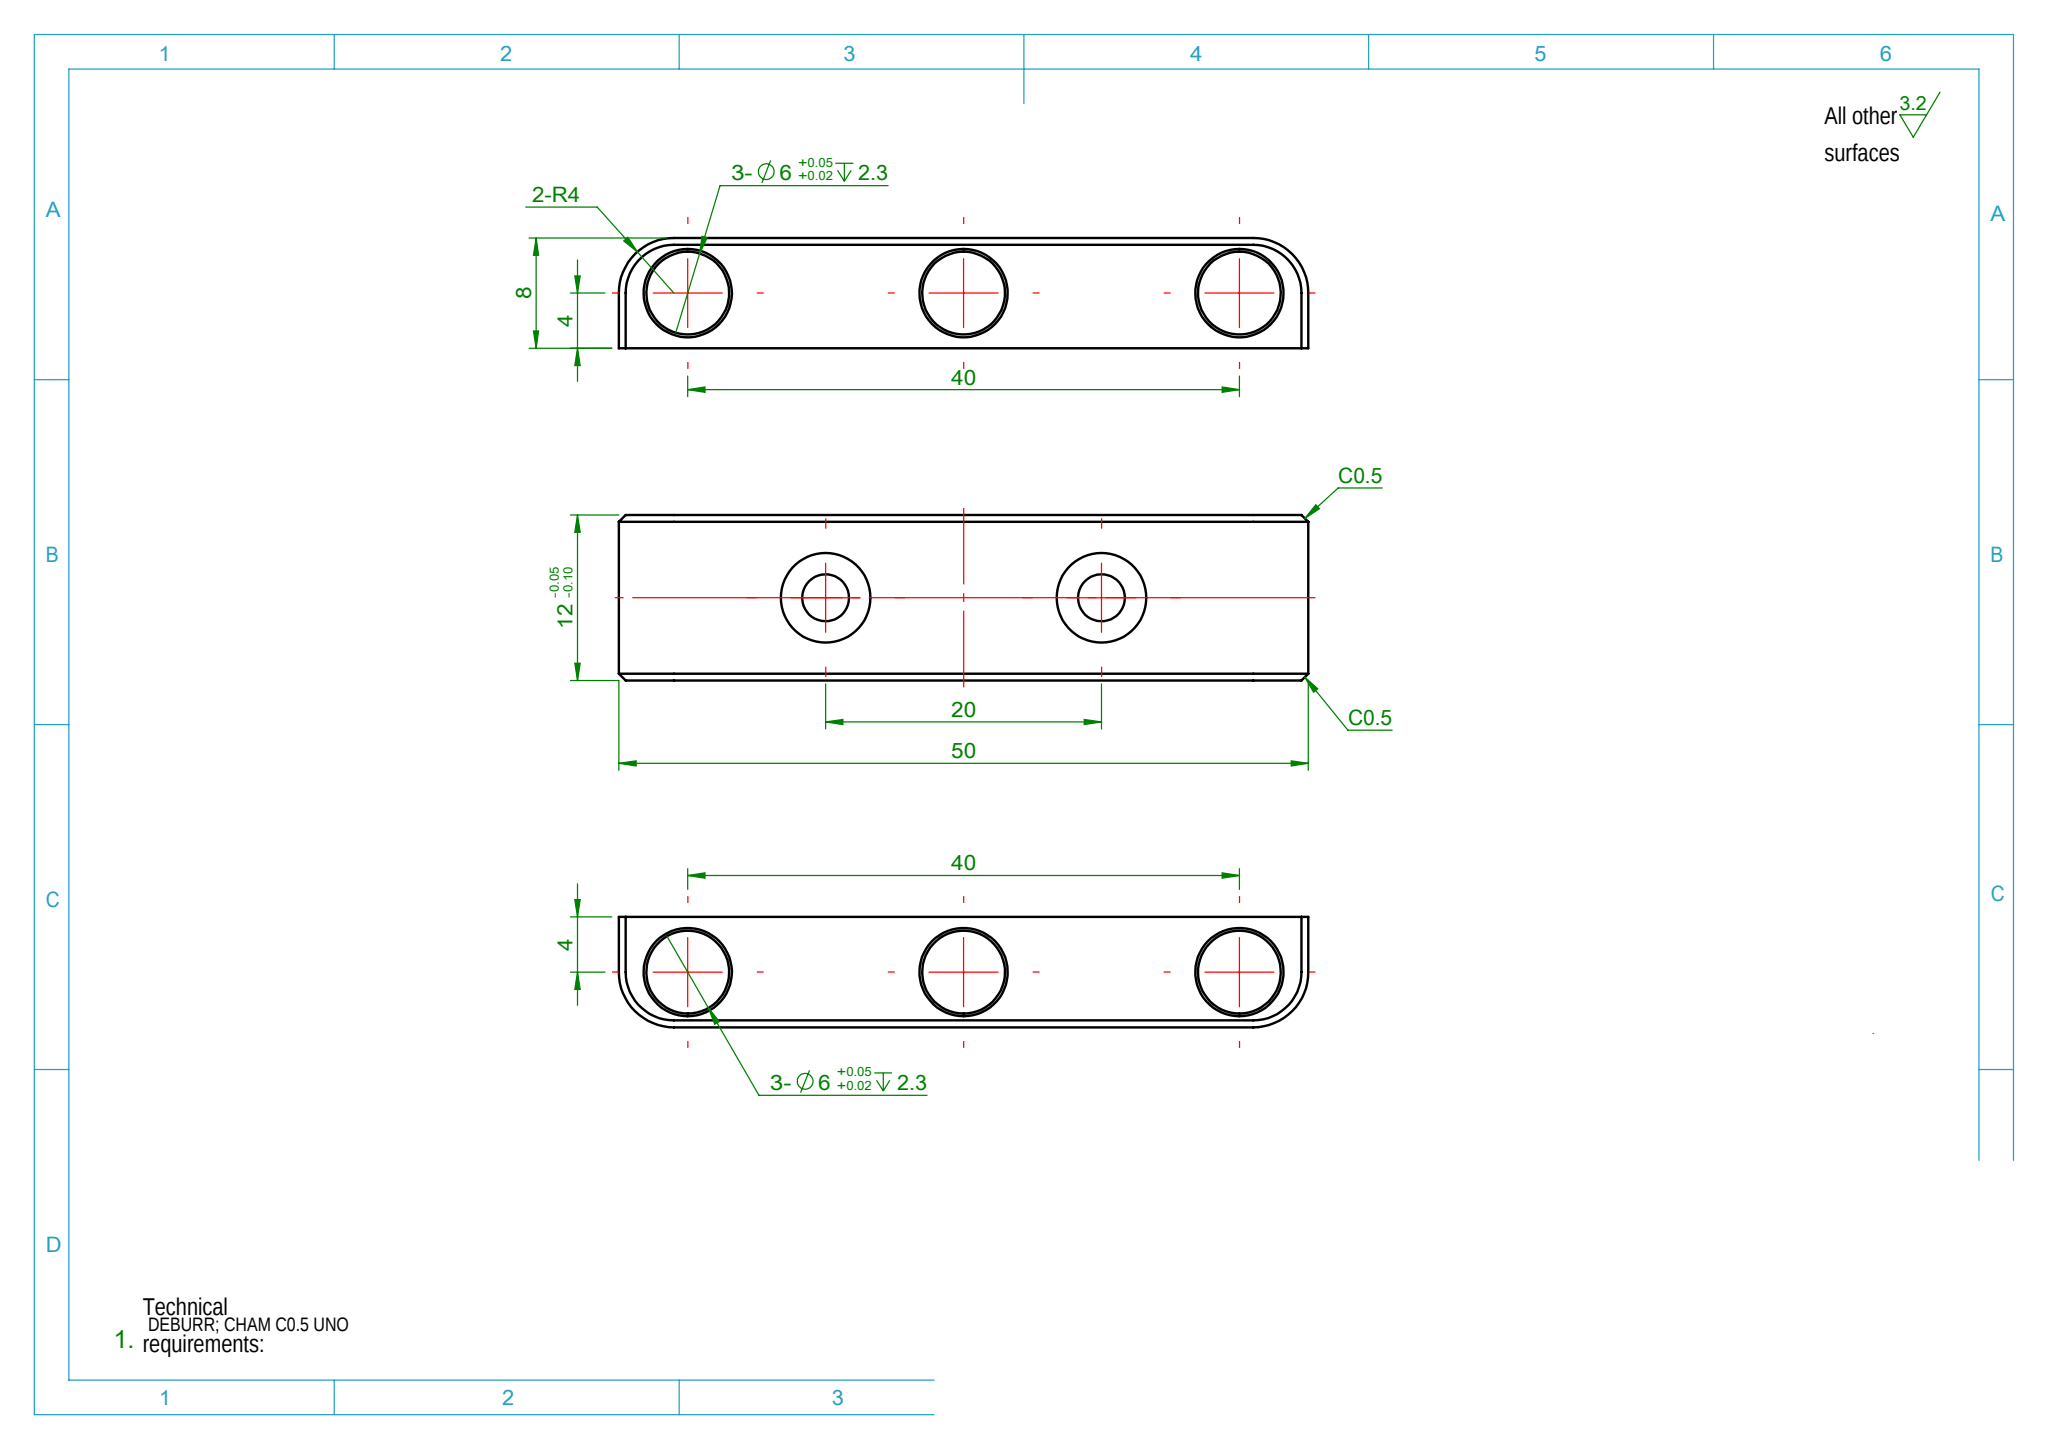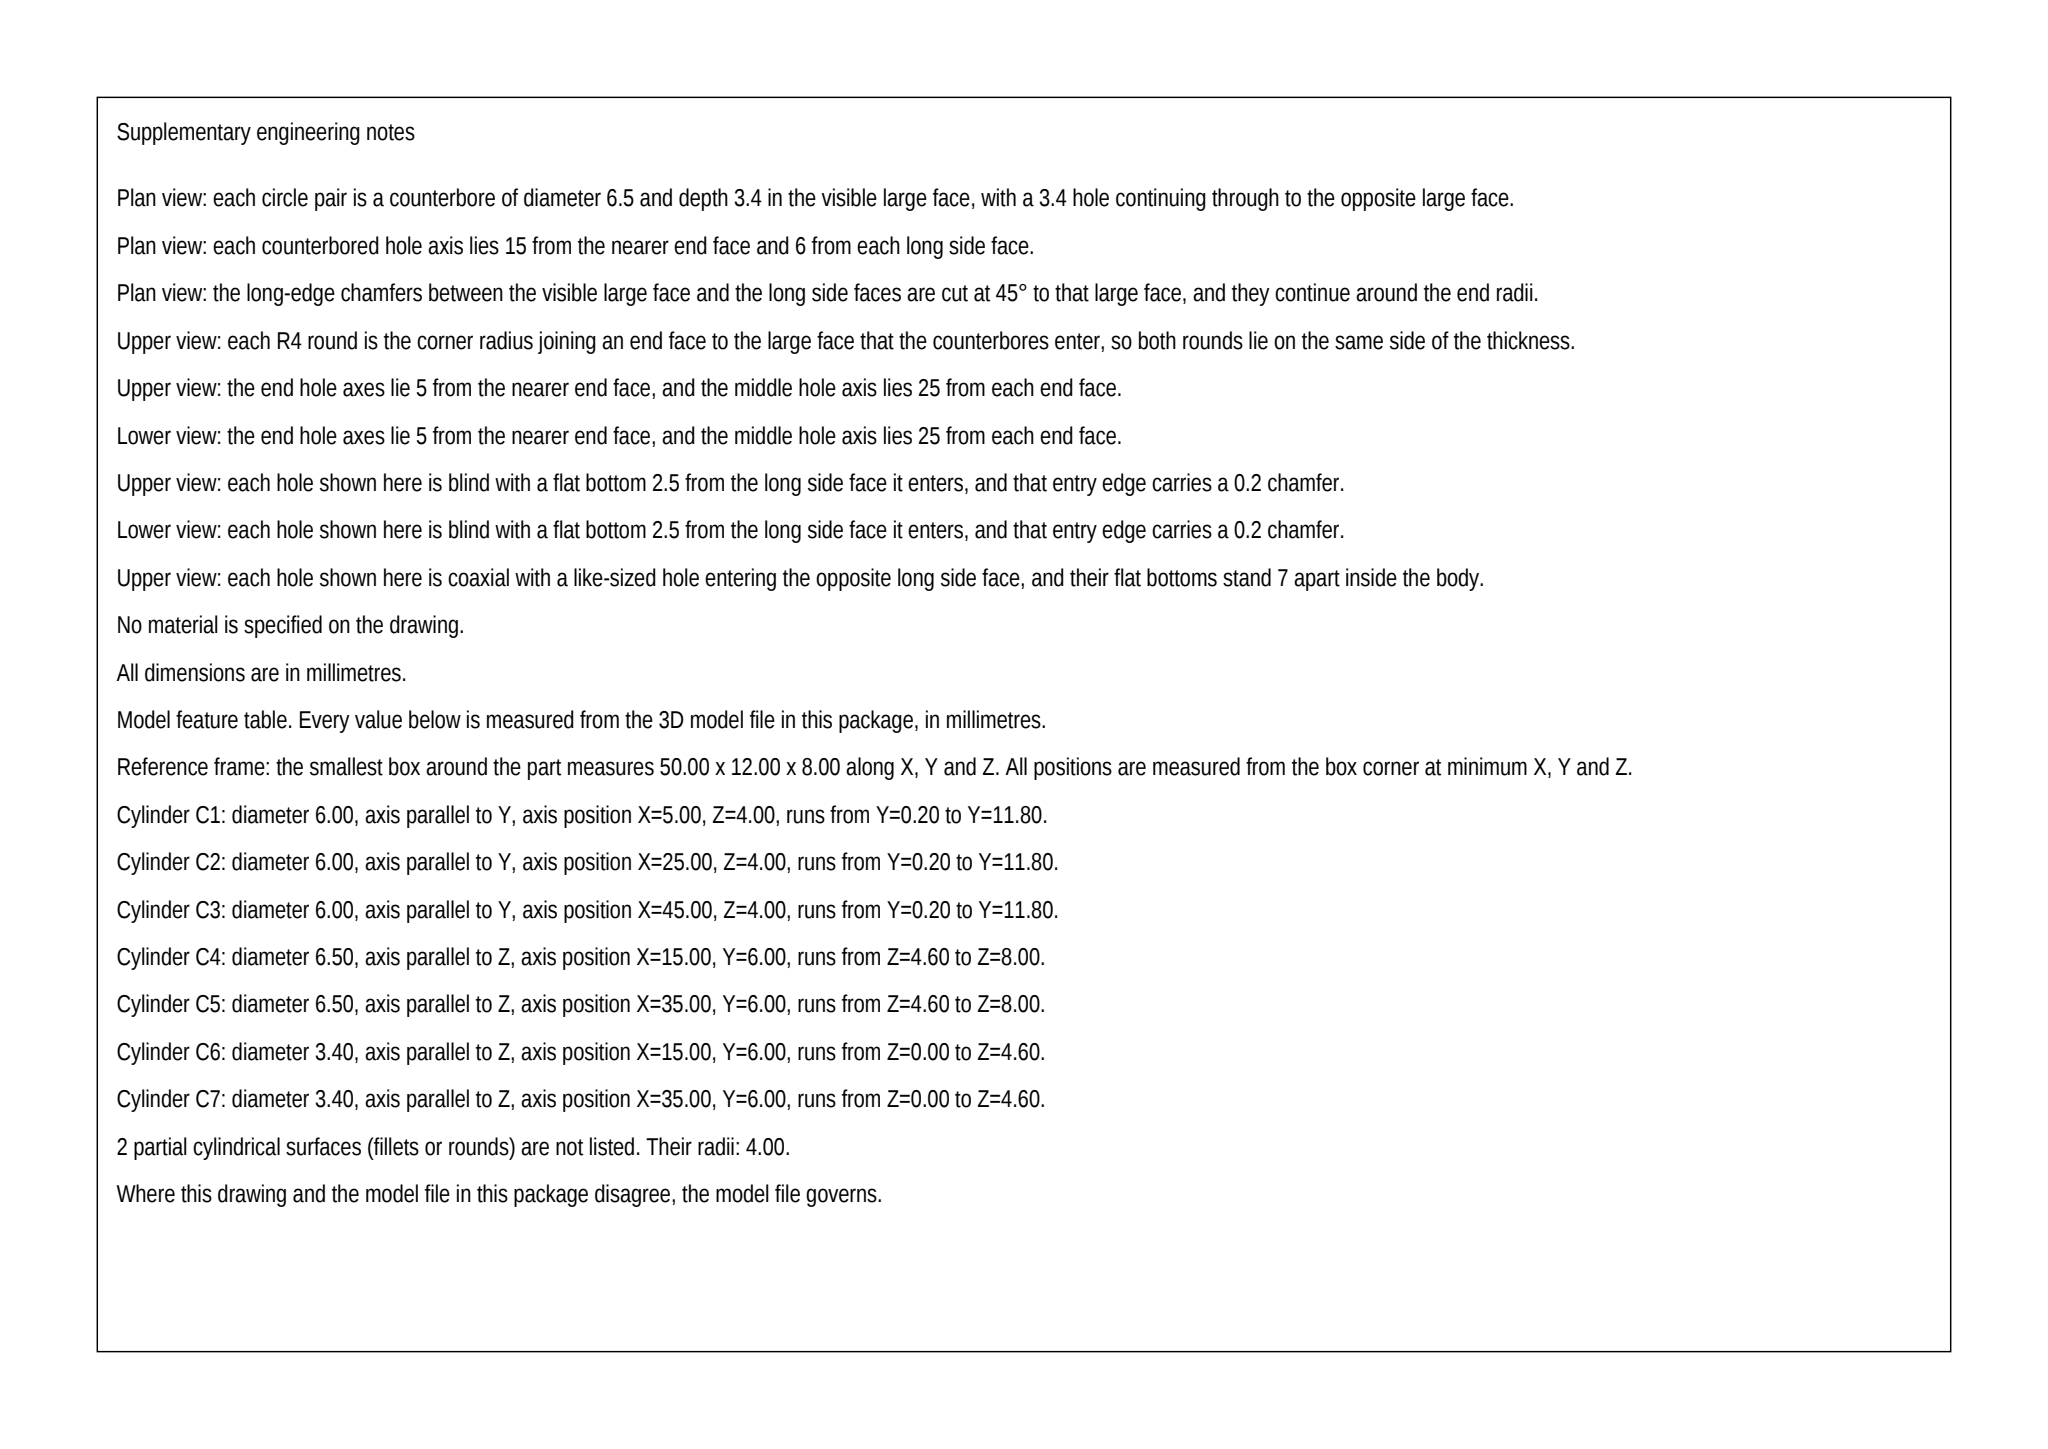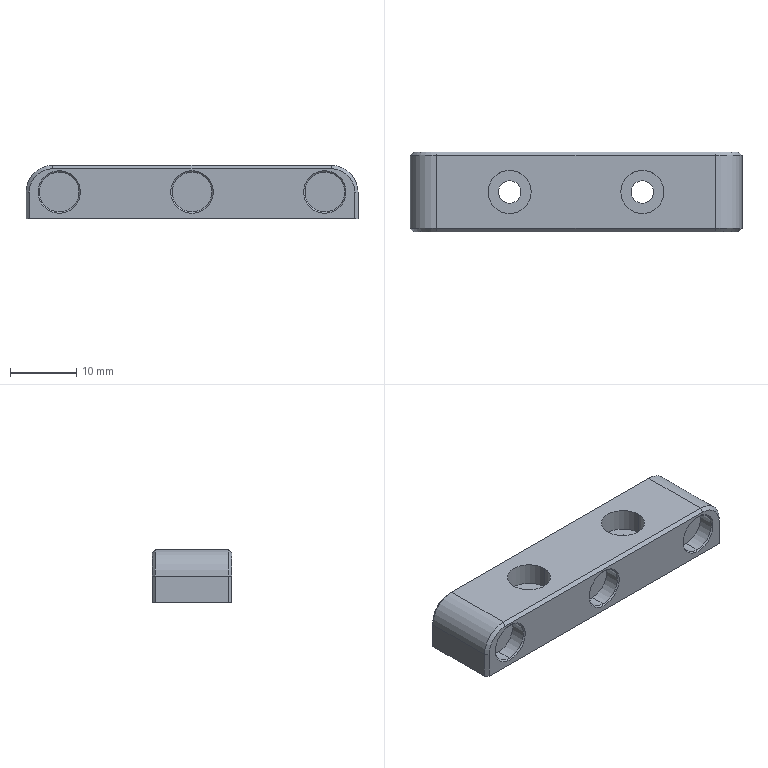Part | SolidWorks | mm | 1 solid | 58 faces | box 50 x 12 x 8 mm | volume 3966 mm3 | cylinder 22 | plane 20 | cone 16 | commonest cylinder face diameters 6 x12 6.5 x4 3.4 x4 8 x2
Drawing notes:
MIDDLE VIEW: 2X Ø3.4 THRU, SPACED 20, ON 12 WIDTH CL | from the solid: cyl dia 3.4 axis z at (15,6) and (35,6), len 4.6 + 3.4 c'bore = 8 thk
2X Ø3.4: CBORE Ø6.5 DP 3.4 FROM TOP FACE | from the solid: cyl dia 6.5 axis z at (15,6),(35,6), len 3.4 from z=4.6 to z=8.0
2X CBORE Ø6.5: CSK 90° X Ø7 AT TOP FACE | from the solid: cones included angle 90.0, ref dia 7.0 at counterbored holes
Ø3.4 THRU (4.6 DP BELOW CBORE ) - 8 TOTAL THK | from the solid: 3.4 cyl len 4.6 from z=0 to 4.6; bbox z=8.0
build123d program:
from build123d import *

# Parameters (mm, degrees)
SKETCH1_W                                       = 80
SKETCH1_H                                       = 8
BOSS_EXTRUDE1_DEPTH                             = 12
SKETCH2_R                                       = 3
CUT_EXTRUDE1_DEPTH                              = 2.5
M3_HEX_SOCKET_HEAD_CAP_SCREW_CBORE1_D           = 3.4
M3_HEX_SOCKET_HEAD_CAP_SCREW_CBORE1_CBORE_D     = 6.5
M3_HEX_SOCKET_HEAD_CAP_SCREW_CBORE1_CBORE_DEPTH = 3.4
CUT_EXTRUDE2_START                              = -2.5
SKETCH7_R                                       = 3
CUT_EXTRUDE2_DEPTH                              = 2.5
CHAMFER1_SIZE                                   = 0.2
SKETCH8_W                                       = 30
SKETCH8_H                                       = 12
CUT_EXTRUDE3_DEPTH                              = 10
FILLET1_R                                       = 4
CHAMFER2_SIZE                                   = 0.5


with BuildPart() as part:
    # Sketch1 → Boss-Extrude1 (new body)
    with BuildSketch(Plane(origin=(0, 0, 0), x_dir=(1, 0, 0), z_dir=(0, 1, 0))):
        with Locations((40, 4)):
            Rectangle(SKETCH1_W, SKETCH1_H)
    extrude(amount=BOSS_EXTRUDE1_DEPTH)

    # Sketch2 → Cut-Extrude1 (cut)
    with BuildSketch(Plane.XZ):
        with Locations(Location((75, -4, 0), (0, 0, 270))):
            Circle(SKETCH2_R)
        with Locations(Location((45, -4, 0), (0, 0, 270))):
            Circle(SKETCH2_R)
        with Locations(Location((25, -4, 0), (0, 0, 270))):
            Circle(SKETCH2_R)
        with Locations(Location((5, -4, 0), (0, 0, 270))):
            Circle(SKETCH2_R)
    extrude(amount=-CUT_EXTRUDE1_DEPTH, mode=Mode.SUBTRACT)

    # M3 Hex Socket Head Cap Screw CBORE1 (through all)
    with Locations(Plane.XY):
        with Locations((15, 6), (35, 6)):
            CounterBoreHole(M3_HEX_SOCKET_HEAD_CAP_SCREW_CBORE1_D / 2, M3_HEX_SOCKET_HEAD_CAP_SCREW_CBORE1_CBORE_D / 2, M3_HEX_SOCKET_HEAD_CAP_SCREW_CBORE1_CBORE_DEPTH)

    # Sketch7 → Cut-Extrude2 (cut)
    with BuildSketch(Plane(origin=(0, 12, 0), x_dir=(1, 0, 0), z_dir=(0, 1, 0)).offset(CUT_EXTRUDE2_START)):
        with Locations(Location((75, 4, 0), (0, 0, 90))):
            Circle(SKETCH7_R)
        with Locations(Location((25, 4, 0), (0, 0, 90))):
            Circle(SKETCH7_R)
        with Locations(Location((45, 4, 0), (0, 0, 90))):
            Circle(SKETCH7_R)
        with Locations(Location((5, 4, 0), (0, 0, 90))):
            Circle(SKETCH7_R)
    extrude(amount=CUT_EXTRUDE2_DEPTH, mode=Mode.SUBTRACT)

    # Chamfer1
    chamfer1_edges = [part.edges().sort_by_distance(p)[0] for p in [
        (75, 0, -1),
        (45, 0, -1),
        (25, 0, -1),
        (5, 0, -1),
        (75, 12, -1),
        (45, 12, -1),
        (25, 12, -1),
        (5, 12, -1),
    ]]
    chamfer(chamfer1_edges, length=CHAMFER1_SIZE)

    # Sketch8 → Cut-Extrude3 (cut)
    with BuildSketch(Plane.XY):
        with Locations((65, 6)):
            Rectangle(SKETCH8_W, SKETCH8_H)
    extrude(amount=-CUT_EXTRUDE3_DEPTH, mode=Mode.SUBTRACT)

    # Fillet1
    fillet1_edges = [part.edges().sort_by_distance(p)[0] for p in [
        (0, 6, 0),
        (50, 6, 0),
    ]]
    fillet(fillet1_edges, radius=FILLET1_R)

    # Chamfer2
    chamfer2_edges = [part.edges().sort_by_distance(p)[0] for p in [
        (25, 0, 0),
        (0, 0, -6),
        (1.172, 0, -1.172),
        (48.828, 0, -1.172),
        (25, 12, 0),
        (0, 12, -6),
        (1.172, 12, -1.172),
        (48.828, 12, -1.172),
        (50, 0, -6),
        (50, 12, -6),
    ]]
    chamfer(chamfer2_edges, length=CHAMFER2_SIZE)


solid = part.part